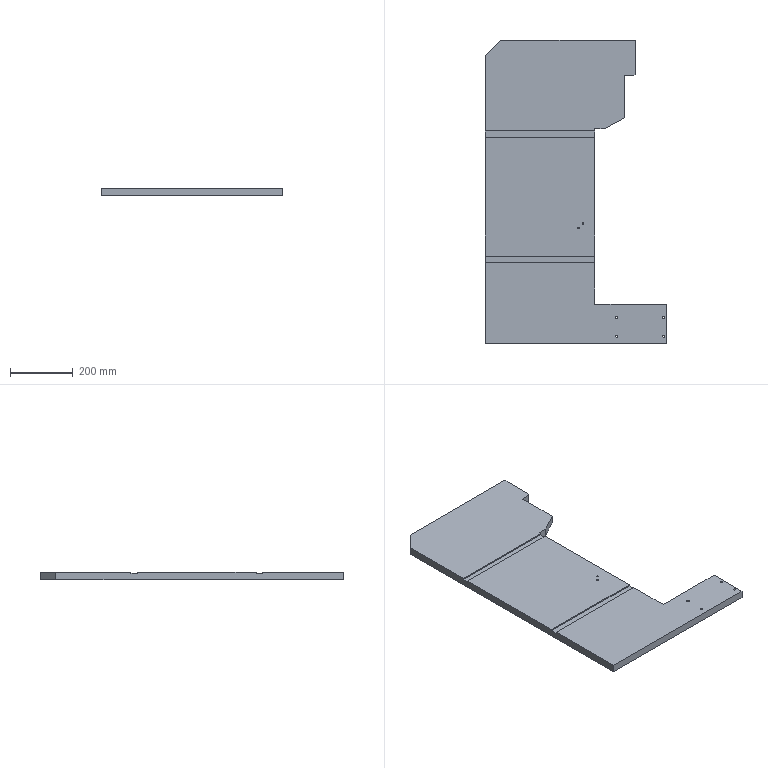Component | SolidWorks | 100-03-1 | 1 solid | 71 faces | box 580 x 970 x 25 mm | volume 9856992 mm3 | cylinder 32 | plane 27 | cone 12 | commonest cylinder face diameters 11 x8 6.6 x8 2.5 x8 6.8 x4 5 x4 | material 45
build123d program:
from build123d import *

# Parameters (mm, degrees)
BOSS_EXTRUDE1_DEPTH                               = 12.5
CHAMFER1_SIZE                                     = 5
M6_TAPPED_HOLE1_D                                 = 5
M3_TAPPED_HOLE1_D                                 = 2.5
M3_TAPPED_HOLE1_DEPTH                             = 7.5
M3_TAPPED_HOLE1_TIP                               = 0.7511
SKETCH11_W                                        = 350
SKETCH11_H                                        = 20
CUT_EXTRUDE1_DEPTH                                = 4
LPATTERN1_COUNT                                   = 2
LPATTERN1_PITCH                                   = 400
M8_TAPPED_HOLE1_D                                 = 6.8
M8_TAPPED_HOLE1_DEPTH                             = 19.75
M8_TAPPED_HOLE1_TIP                               = 2.043
HOLE_SIZE_ACCORDING_TO_HEXAGON_SOCKET_D           = 6.6
HOLE_SIZE_ACCORDING_TO_HEXAGON_SOCKET_CBORE_D     = 11
HOLE_SIZE_ACCORDING_TO_HEXAGON_SOCKET_CBORE_DEPTH = 4.7


with BuildPart() as part:
    # Sketch1 → Boss-Extrude1 (new, symmetric)
    with BuildSketch(Plane.XY):
        Polygon((580, 126), (350, 126), (350, 687), (380, 687), (445, 722), (445, 857), (479, 857), (479, 970), (50, 970), (0, 920), (0, 0), (580, 0), align=None)
    extrude(amount=BOSS_EXTRUDE1_DEPTH, both=True)

    # Chamfer1
    chamfer1_edges = [part.edges().sort_by_distance(p)[0] for p in [
        (479, 857, 0),
    ]]
    chamfer(chamfer1_edges, length=CHAMFER1_SIZE)

    # M6 Tapped Hole1 (through all)
    with Locations(Plane(origin=(0, 0, -12.5), x_dir=(-1, 0, 0), z_dir=(0, 0, -1))):
        with Locations((-298, 370), (-312.142, 384.142)):
            Hole(M6_TAPPED_HOLE1_D / 2)

    # M3 Tapped Hole1
    with Locations(Plane(origin=(0, 0, -12.5), x_dir=(-1, 0, 0), z_dir=(0, 0, -1))):
        with Locations((-145, 354), (-60, 354), (-145, 320), (-60, 320)):
            Hole(M3_TAPPED_HOLE1_D / 2, depth=M3_TAPPED_HOLE1_DEPTH)
            with Locations((0, 0, -(M3_TAPPED_HOLE1_DEPTH + M3_TAPPED_HOLE1_TIP / 2))):  # 118° drill point
                Cone(0, M3_TAPPED_HOLE1_D / 2, M3_TAPPED_HOLE1_TIP, mode=Mode.SUBTRACT)

    # Sketch11 → Cut-Extrude1 (cut)
    with BuildSketch(Plane.XY.offset(12.5)):
        with Locations((175, 270)):
            Rectangle(SKETCH11_W, SKETCH11_H)
    cut_extrude1 = extrude(amount=-CUT_EXTRUDE1_DEPTH, mode=Mode.SUBTRACT)

    # LPattern1: Cut-Extrude1 ×2
    with Locations(*[(0, i * LPATTERN1_PITCH, 0) for i in range(1, LPATTERN1_COUNT)]):
        add(cut_extrude1, mode=Mode.SUBTRACT)

    # M8 Tapped Hole1
    with Locations(Plane(origin=(0, 126, 0), x_dir=(1, 0, 0), z_dir=(0, 1, 0))):
        with Locations((552.5, 0), (507.5, 0)):
            Hole(M8_TAPPED_HOLE1_D / 2, depth=M8_TAPPED_HOLE1_DEPTH)
            with Locations((0, 0, -(M8_TAPPED_HOLE1_DEPTH + M8_TAPPED_HOLE1_TIP / 2))):  # 118° drill point
                Cone(0, M8_TAPPED_HOLE1_D / 2, M8_TAPPED_HOLE1_TIP, mode=Mode.SUBTRACT)

    # Hole Size _According to_ Hexagon Socket (through all)
    with Locations(Plane(origin=(0, 0, -12.5), x_dir=(-1, 0, 0), z_dir=(0, 0, -1))):
        with Locations((-570, 24), (-570, 84), (-420, 24), (-420, 84)):
            CounterBoreHole(HOLE_SIZE_ACCORDING_TO_HEXAGON_SOCKET_D / 2, HOLE_SIZE_ACCORDING_TO_HEXAGON_SOCKET_CBORE_D / 2, HOLE_SIZE_ACCORDING_TO_HEXAGON_SOCKET_CBORE_DEPTH)


solid = part.part

# Placed as in the assembly
solid = solid.moved(Location((-300, 14, -97.5), (0, 0, 0)))